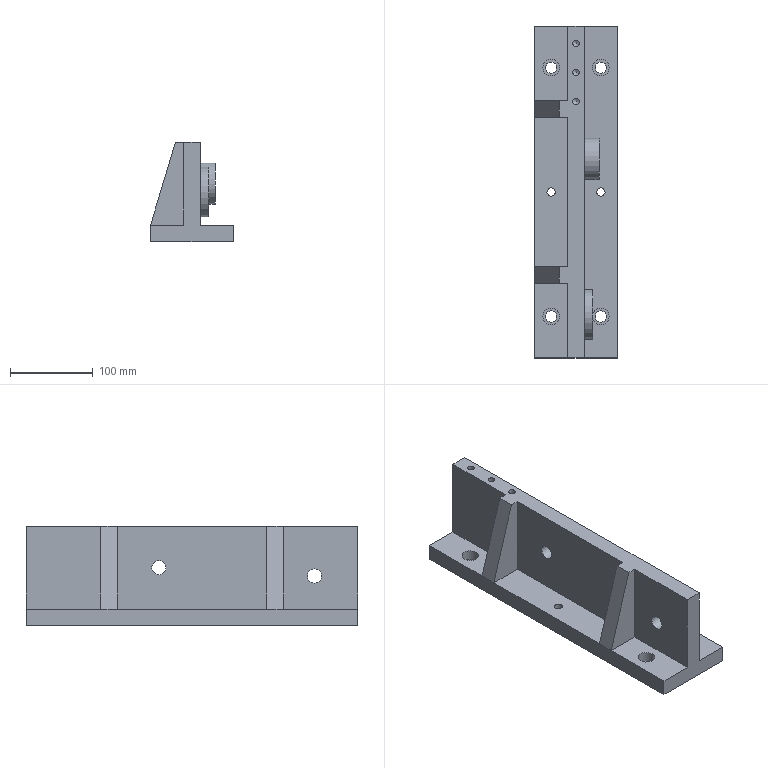Component | NX | FIXTURE_BODY | 1 solid | 46 faces | volume 1722387 mm3 | plane 26 | cylinder 17 | cone 3 | commonest cylinder face diameters 13.5 x4 20 x4 8 x3 17 x2 10 x2 60 x1 50 x1